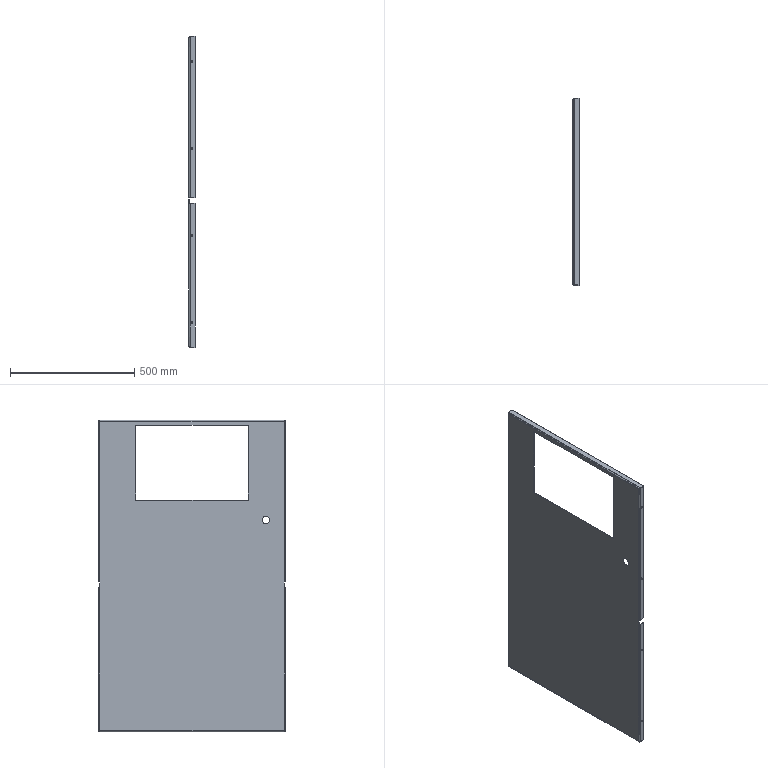Component | SolidWorks | Partition(No.50)-1 | 1 solid | 76 faces | volume 1770180 mm3 | plane 38 | cylinder 30 | spline 8 | commonest cylinder face diameters 6.5 x16 10 x6 6 x6 30 x2 | material Plain Carbon Steel